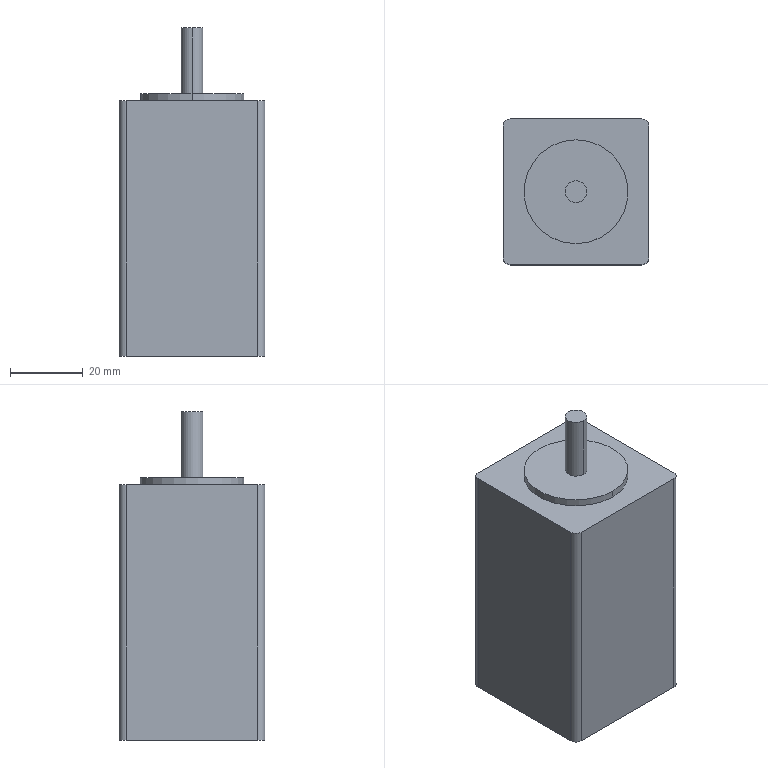Component | SolidWorks | Motor-1 | 1 solid | 16 faces | box 40 x 40 x 90 mm | volume 113537 mm3 | cylinder 8 | plane 8 | commonest cylinder face diameters 4 x4 5.952 x2 28.506 x2
build123d program:
from build123d import *

# Parameters (mm, degrees)
SKETCH1_W           = 40
SKETCH1_H           = 70
BOSS_EXTRUDE1_DEPTH = 40
FILLET1_R           = 2
BOSS_EXTRUDE2_DEPTH = 2
SKETCH3_R           = 2.976
BOSS_EXTRUDE3_DEPTH = 18


with BuildPart() as part:
    # Sketch1 → Boss-Extrude1 (new body)
    with BuildSketch(Plane.XY):
        with Locations((59.88, -78.689)):
            Rectangle(SKETCH1_W, SKETCH1_H)
    extrude(amount=BOSS_EXTRUDE1_DEPTH)

    # Fillet1
    fillet1_edges = [part.edges().sort_by_distance(p)[0] for p in [
        (79.88, -78.689, 40),
        (39.88, -78.689, 40),
        (79.88, -78.689, 0),
        (39.88, -78.689, 0),
    ]]
    fillet(fillet1_edges, radius=FILLET1_R)

    # Sketch2 → Boss-Extrude2 (add)
    with BuildSketch(Plane(origin=(0, -43.689, 0), x_dir=(1, 0, 0), z_dir=(0, 1, 0))):
        with BuildLine():
            ThreePointArc((59.88, -5.747), (45.627, -20), (59.88, -34.253))
            Line((59.88, -34.253), (59.88, -5.747))
        make_face()
        with BuildLine():
            Line((59.88, -5.747), (59.88, -34.253))
            ThreePointArc((59.88, -34.253), (69.959, -30.078), (74.133, -20))
            ThreePointArc((74.133, -20), (69.959, -9.922), (59.88, -5.747))
        make_face()
        with BuildLine():
            ThreePointArc((59.88, -5.747), (45.627, -20), (59.88, -34.253))
            Line((59.88, -34.253), (59.88, -5.747))
        make_face()
        with BuildLine():
            Line((59.88, -5.747), (59.88, -34.253))
            ThreePointArc((59.88, -34.253), (69.959, -30.078), (74.133, -20))
            ThreePointArc((74.133, -20), (69.959, -9.922), (59.88, -5.747))
        make_face()
    extrude(amount=BOSS_EXTRUDE2_DEPTH)

    # Sketch3 → Boss-Extrude3 (add)
    with BuildSketch(Plane(origin=(0, -41.689, 0), x_dir=(1, 0, 0), z_dir=(0, 1, 0))):
        with Locations(Location((59.88, -20, 0), (0, 0, 270))):
            Circle(SKETCH3_R)
    extrude(amount=BOSS_EXTRUDE3_DEPTH)


solid = part.part

# Placed as in the assembly
solid = solid.moved(Location((-11.374, -44.609, -171.311), (90, 0, 0)))
STEP:
#1=CARTESIAN_POINT('',(1.91,-2.661,-7.677));
#2=VERTEX_POINT('',#1);
#3=CARTESIAN_POINT('',(1.91,-2.426,-7.677));
#4=VERTEX_POINT('',#3);
#5=CARTESIAN_POINT('',(1.91,-2.544,-7.677));
#6=DIRECTION('',(0.,0.,1.));
#7=DIRECTION('',(0.,-1.,0.));
#8=AXIS2_PLACEMENT_3D('',#5,#6,#7);
#9=CIRCLE('',#8,0.1172);
#10=EDGE_CURVE('',#2,#4,#9,.T.);
#11=ORIENTED_EDGE('',*,*,#10,.F.);
#12=CARTESIAN_POINT('',(1.91,-2.661,-8.386));
#13=VERTEX_POINT('',#12);
#14=CARTESIAN_POINT('',(1.91,-2.661,-7.677));
#15=DIRECTION('',(0.,0.,-1.));
#16=VECTOR('',#15,39.37);
#17=LINE('',#14,#16);
#18=EDGE_CURVE('',#2,#13,#17,.T.);
#19=ORIENTED_EDGE('',*,*,#18,.T.);
#20=CARTESIAN_POINT('',(1.91,-2.426,-8.386));
#21=VERTEX_POINT('',#20);
#22=CARTESIAN_POINT('',(1.91,-2.544,-8.386));
#23=DIRECTION('',(0.,0.,1.));
#24=DIRECTION('',(0.,-1.,0.));
#25=AXIS2_PLACEMENT_3D('',#22,#23,#24);
#26=CIRCLE('',#25,0.1172);
#27=EDGE_CURVE('',#13,#21,#26,.T.);
#28=ORIENTED_EDGE('',*,*,#27,.T.);
#29=CARTESIAN_POINT('',(1.91,-2.426,-7.677));
#30=DIRECTION('',(0.,0.,-1.));
#31=VECTOR('',#30,39.37);
#32=LINE('',#29,#31);
#33=EDGE_CURVE('',#4,#21,#32,.T.);
#34=ORIENTED_EDGE('',*,*,#33,.F.);
#35=EDGE_LOOP('',(#11,#19,#28,#34));
#36=FACE_OUTER_BOUND('',#35,.T.);
#37=CARTESIAN_POINT('',(1.91,-2.544,-7.677));
#38=DIRECTION('',(0.,0.,-1.));
#39=DIRECTION('',(0.,1.,0.));
#40=AXIS2_PLACEMENT_3D('',#37,#38,#39);
#41=CYLINDRICAL_SURFACE('',#40,0.1172);
#42=ADVANCED_FACE('',(#36),#41,.T.);
#43=CARTESIAN_POINT('',(1.91,-3.105,-8.386));
#44=VERTEX_POINT('',#43);
#45=CARTESIAN_POINT('',(1.91,-1.983,-8.386));
#46=VERTEX_POINT('',#45);
#47=CARTESIAN_POINT('',(1.91,-2.544,-8.386));
#48=DIRECTION('',(0.,0.,1.));
#49=DIRECTION('',(0.,-1.,0.));
#50=AXIS2_PLACEMENT_3D('',#47,#48,#49);
#51=CIRCLE('',#50,0.5611);
#52=EDGE_CURVE('',#44,#46,#51,.T.);
#53=ORIENTED_EDGE('',*,*,#52,.F.);
#54=CARTESIAN_POINT('',(1.91,-3.105,-8.465));
#55=VERTEX_POINT('',#54);
#56=CARTESIAN_POINT('',(1.91,-3.105,-8.386));
#57=DIRECTION('',(0.,0.,-1.));
#58=VECTOR('',#57,39.37);
#59=LINE('',#56,#58);
#60=EDGE_CURVE('',#44,#55,#59,.T.);
#61=ORIENTED_EDGE('',*,*,#60,.T.);
#62=CARTESIAN_POINT('',(1.91,-1.983,-8.465));
#63=VERTEX_POINT('',#62);
#64=CARTESIAN_POINT('',(1.91,-2.544,-8.465));
#65=DIRECTION('',(0.,0.,1.));
#66=DIRECTION('',(0.,-1.,0.));
#67=AXIS2_PLACEMENT_3D('',#64,#65,#66);
#68=CIRCLE('',#67,0.5611);
#69=EDGE_CURVE('',#55,#63,#68,.T.);
#70=ORIENTED_EDGE('',*,*,#69,.T.);
#71=CARTESIAN_POINT('',(1.91,-1.983,-8.386));
#72=DIRECTION('',(0.,0.,-1.));
#73=VECTOR('',#72,39.37);
#74=LINE('',#71,#73);
#75=EDGE_CURVE('',#46,#63,#74,.T.);
#76=ORIENTED_EDGE('',*,*,#75,.F.);
#77=EDGE_LOOP('',(#53,#61,#70,#76));
#78=FACE_OUTER_BOUND('',#77,.T.);
#79=CARTESIAN_POINT('',(1.91,-2.544,-8.386));
#80=DIRECTION('',(0.,0.,-1.));
#81=DIRECTION('',(0.,1.,0.));
#82=AXIS2_PLACEMENT_3D('',#79,#80,#81);
#83=CYLINDRICAL_SURFACE('',#82,0.5611);
#84=ADVANCED_FACE('',(#78),#83,.T.);
#85=CARTESIAN_POINT('',(1.122,-3.252,-8.465));
#86=VERTEX_POINT('',#85);
#87=CARTESIAN_POINT('',(1.122,-1.835,-8.465));
#88=VERTEX_POINT('',#87);
#89=CARTESIAN_POINT('',(1.122,-3.331,-8.465));
#90=DIRECTION('',(0.,1.,0.));
#91=VECTOR('',#90,39.37);
#92=LINE('',#89,#91);
#93=EDGE_CURVE('',#86,#88,#92,.T.);
#94=ORIENTED_EDGE('',*,*,#93,.T.);
#95=CARTESIAN_POINT('',(1.122,-1.835,-11.22));
#96=VERTEX_POINT('',#95);
#97=CARTESIAN_POINT('',(1.122,-1.835,-8.465));
#98=DIRECTION('',(0.,0.,-1.));
#99=VECTOR('',#98,39.37);
#100=LINE('',#97,#99);
#101=EDGE_CURVE('',#88,#96,#100,.T.);
#102=ORIENTED_EDGE('',*,*,#101,.T.);
#103=CARTESIAN_POINT('',(1.122,-3.252,-11.22));
#104=VERTEX_POINT('',#103);
#105=CARTESIAN_POINT('',(1.122,-3.331,-11.22));
#106=DIRECTION('',(0.,1.,0.));
#107=VECTOR('',#106,39.37);
#108=LINE('',#105,#107);
#109=EDGE_CURVE('',#104,#96,#108,.T.);
#110=ORIENTED_EDGE('',*,*,#109,.F.);
#111=CARTESIAN_POINT('',(1.122,-3.252,-8.465));
#112=DIRECTION('',(-0.,0.,1.));
#113=VECTOR('',#112,39.37);
#114=LINE('',#111,#113);
#115=EDGE_CURVE('',#104,#86,#114,.T.);
#116=ORIENTED_EDGE('',*,*,#115,.T.);
#117=EDGE_LOOP('',(#94,#102,#110,#116));
#118=FACE_OUTER_BOUND('',#117,.T.);
#119=CARTESIAN_POINT('',(1.122,-3.331,-8.465));
#120=DIRECTION('',(1.,0.,0.));
#121=DIRECTION('',(-0.,0.,1.));
#122=AXIS2_PLACEMENT_3D('',#119,#120,#121);
#123=PLANE('',#122);
#124=ADVANCED_FACE('',(#118),#123,.F.);
#125=CARTESIAN_POINT('',(1.201,-1.756,-11.22));
#126=VERTEX_POINT('',#125);
#127=CARTESIAN_POINT('',(2.618,-1.756,-11.22));
#128=VERTEX_POINT('',#127);
#129=CARTESIAN_POINT('',(1.122,-1.756,-11.22));
#130=DIRECTION('',(1.,0.,0.));
#131=VECTOR('',#130,39.37);
#132=LINE('',#129,#131);
#133=EDGE_CURVE('',#126,#128,#132,.T.);
#134=ORIENTED_EDGE('',*,*,#133,.T.);
#135=CARTESIAN_POINT('',(2.697,-1.835,-11.22));
#136=VERTEX_POINT('',#135);
#137=CARTESIAN_POINT('',(2.618,-1.835,-11.22));
#138=DIRECTION('',(0.,0.,-1.));
#139=DIRECTION('',(0.,-1.,0.));
#140=AXIS2_PLACEMENT_3D('',#137,#138,#139);
#141=CIRCLE('',#140,0.07874);
#142=EDGE_CURVE('',#128,#136,#141,.T.);
#143=ORIENTED_EDGE('',*,*,#142,.T.);
#144=CARTESIAN_POINT('',(2.697,-3.252,-11.22));
#145=VERTEX_POINT('',#144);
#146=CARTESIAN_POINT('',(2.697,-3.331,-11.22));
#147=DIRECTION('',(0.,1.,0.));
#148=VECTOR('',#147,39.37);
#149=LINE('',#146,#148);
#150=EDGE_CURVE('',#145,#136,#149,.T.);
#151=ORIENTED_EDGE('',*,*,#150,.F.);
#152=CARTESIAN_POINT('',(2.618,-3.331,-11.22));
#153=VERTEX_POINT('',#152);
#154=CARTESIAN_POINT('',(2.618,-3.252,-11.22));
#155=DIRECTION('',(0.,0.,-1.));
#156=DIRECTION('',(0.,-1.,0.));
#157=AXIS2_PLACEMENT_3D('',#154,#155,#156);
#158=CIRCLE('',#157,0.07874);
#159=EDGE_CURVE('',#145,#153,#158,.T.);
#160=ORIENTED_EDGE('',*,*,#159,.T.);
#161=CARTESIAN_POINT('',(1.201,-3.331,-11.22));
#162=VERTEX_POINT('',#161);
#163=CARTESIAN_POINT('',(1.122,-3.331,-11.22));
#164=DIRECTION('',(1.,0.,0.));
#165=VECTOR('',#164,39.37);
#166=LINE('',#163,#165);
#167=EDGE_CURVE('',#162,#153,#166,.T.);
#168=ORIENTED_EDGE('',*,*,#167,.F.);
#169=CARTESIAN_POINT('',(1.201,-3.252,-11.22));
#170=DIRECTION('',(0.,0.,-1.));
#171=DIRECTION('',(0.,-1.,0.));
#172=AXIS2_PLACEMENT_3D('',#169,#170,#171);
#173=CIRCLE('',#172,0.07874);
#174=EDGE_CURVE('',#162,#104,#173,.T.);
#175=ORIENTED_EDGE('',*,*,#174,.T.);
#176=ORIENTED_EDGE('',*,*,#109,.T.);
#177=CARTESIAN_POINT('',(1.201,-1.835,-11.22));
#178=DIRECTION('',(0.,0.,-1.));
#179=DIRECTION('',(0.,-1.,0.));
#180=AXIS2_PLACEMENT_3D('',#177,#178,#179);
#181=CIRCLE('',#180,0.07874);
#182=EDGE_CURVE('',#96,#126,#181,.T.);
#183=ORIENTED_EDGE('',*,*,#182,.T.);
#184=EDGE_LOOP('',(#134,#143,#151,#160,#168,#175,#176,#183));
#185=FACE_OUTER_BOUND('',#184,.T.);
#186=CARTESIAN_POINT('',(1.122,-3.331,-11.22));
#187=DIRECTION('',(0.,0.,1.));
#188=DIRECTION('',(0.,-1.,0.));
#189=AXIS2_PLACEMENT_3D('',#186,#187,#188);
#190=PLANE('',#189);
#191=ADVANCED_FACE('',(#185),#190,.F.);
#192=ORIENTED_EDGE('',*,*,#150,.T.);
#193=CARTESIAN_POINT('',(2.697,-1.835,-8.465));
#194=VERTEX_POINT('',#193);
#195=CARTESIAN_POINT('',(2.697,-1.835,-8.465));
#196=DIRECTION('',(0.,0.,1.));
#197=VECTOR('',#196,39.37);
#198=LINE('',#195,#197);
#199=EDGE_CURVE('',#136,#194,#198,.T.);
#200=ORIENTED_EDGE('',*,*,#199,.T.);
#201=CARTESIAN_POINT('',(2.697,-3.252,-8.465));
#202=VERTEX_POINT('',#201);
#203=CARTESIAN_POINT('',(2.697,-3.331,-8.465));
#204=DIRECTION('',(0.,1.,0.));
#205=VECTOR('',#204,39.37);
#206=LINE('',#203,#205);
#207=EDGE_CURVE('',#202,#194,#206,.T.);
#208=ORIENTED_EDGE('',*,*,#207,.F.);
#209=CARTESIAN_POINT('',(2.697,-3.252,-11.22));
#210=DIRECTION('',(0.,0.,-1.));
#211=VECTOR('',#210,39.37);
#212=LINE('',#209,#211);
#213=EDGE_CURVE('',#202,#145,#212,.T.);
#214=ORIENTED_EDGE('',*,*,#213,.T.);
#215=EDGE_LOOP('',(#192,#200,#208,#214));
#216=FACE_OUTER_BOUND('',#215,.T.);
#217=CARTESIAN_POINT('',(2.697,-3.331,-8.465));
#218=DIRECTION('',(-1.,0.,0.));
#219=DIRECTION('',(0.,-1.,0.));
#220=AXIS2_PLACEMENT_3D('',#217,#218,#219);
#221=PLANE('',#220);
#222=ADVANCED_FACE('',(#216),#221,.F.);
#223=CARTESIAN_POINT('',(1.91,-2.544,-8.465));
#224=DIRECTION('',(0.,0.,1.));
#225=DIRECTION('',(0.,-1.,0.));
#226=AXIS2_PLACEMENT_3D('',#223,#224,#225);
#227=CIRCLE('',#226,0.5611);
#228=EDGE_CURVE('',#63,#55,#227,.T.);
#229=ORIENTED_EDGE('',*,*,#228,.F.);
#230=ORIENTED_EDGE('',*,*,#69,.F.);
#231=EDGE_LOOP('',(#229,#230));
#232=FACE_BOUND('',#231,.T.);
#233=ORIENTED_EDGE('',*,*,#207,.T.);
#234=CARTESIAN_POINT('',(2.618,-1.756,-8.465));
#235=VERTEX_POINT('',#234);
#236=CARTESIAN_POINT('',(2.618,-1.835,-8.465));
#237=DIRECTION('',(0.,0.,1.));
#238=DIRECTION('',(0.,1.,0.));
#239=AXIS2_PLACEMENT_3D('',#236,#237,#238);
#240=CIRCLE('',#239,0.07874);
#241=EDGE_CURVE('',#194,#235,#240,.T.);
#242=ORIENTED_EDGE('',*,*,#241,.T.);
#243=CARTESIAN_POINT('',(1.201,-1.756,-8.465));
#244=VERTEX_POINT('',#243);
#245=CARTESIAN_POINT('',(1.122,-1.756,-8.465));
#246=DIRECTION('',(-1.,0.,0.));
#247=VECTOR('',#246,39.37);
#248=LINE('',#245,#247);
#249=EDGE_CURVE('',#235,#244,#248,.T.);
#250=ORIENTED_EDGE('',*,*,#249,.T.);
#251=CARTESIAN_POINT('',(1.201,-1.835,-8.465));
#252=DIRECTION('',(0.,0.,1.));
#253=DIRECTION('',(0.,1.,0.));
#254=AXIS2_PLACEMENT_3D('',#251,#252,#253);
#255=CIRCLE('',#254,0.07874);
#256=EDGE_CURVE('',#244,#88,#255,.T.);
#257=ORIENTED_EDGE('',*,*,#256,.T.);
#258=ORIENTED_EDGE('',*,*,#93,.F.);
#259=CARTESIAN_POINT('',(1.201,-3.331,-8.465));
#260=VERTEX_POINT('',#259);
#261=CARTESIAN_POINT('',(1.201,-3.252,-8.465));
#262=DIRECTION('',(0.,0.,1.));
#263=DIRECTION('',(0.,1.,0.));
#264=AXIS2_PLACEMENT_3D('',#261,#262,#263);
#265=CIRCLE('',#264,0.07874);
#266=EDGE_CURVE('',#86,#260,#265,.T.);
#267=ORIENTED_EDGE('',*,*,#266,.T.);
#268=CARTESIAN_POINT('',(2.618,-3.331,-8.465));
#269=VERTEX_POINT('',#268);
#270=CARTESIAN_POINT('',(1.122,-3.331,-8.465));
#271=DIRECTION('',(-1.,0.,0.));
#272=VECTOR('',#271,39.37);
#273=LINE('',#270,#272);
#274=EDGE_CURVE('',#269,#260,#273,.T.);
#275=ORIENTED_EDGE('',*,*,#274,.F.);
#276=CARTESIAN_POINT('',(2.618,-3.252,-8.465));
#277=DIRECTION('',(0.,0.,1.));
#278=DIRECTION('',(0.,1.,0.));
#279=AXIS2_PLACEMENT_3D('',#276,#277,#278);
#280=CIRCLE('',#279,0.07874);
#281=EDGE_CURVE('',#269,#202,#280,.T.);
#282=ORIENTED_EDGE('',*,*,#281,.T.);
#283=EDGE_LOOP('',(#233,#242,#250,#257,#258,#267,#275,#282));
#284=FACE_OUTER_BOUND('',#283,.T.);
#285=CARTESIAN_POINT('',(1.122,-3.331,-8.465));
#286=DIRECTION('',(0.,0.,-1.));
#287=DIRECTION('',(0.,1.,0.));
#288=AXIS2_PLACEMENT_3D('',#285,#286,#287);
#289=PLANE('',#288);
#290=ADVANCED_FACE('',(#232,#284),#289,.F.);
#291=ORIENTED_EDGE('',*,*,#274,.T.);
#292=CARTESIAN_POINT('',(1.201,-3.331,-11.22));
#293=DIRECTION('',(0.,0.,-1.));
#294=VECTOR('',#293,39.37);
#295=LINE('',#292,#294);
#296=EDGE_CURVE('',#260,#162,#295,.T.);
#297=ORIENTED_EDGE('',*,*,#296,.T.);
#298=ORIENTED_EDGE('',*,*,#167,.T.);
#299=CARTESIAN_POINT('',(2.618,-3.331,-8.465));
#300=DIRECTION('',(0.,0.,1.));
#301=VECTOR('',#300,39.37);
#302=LINE('',#299,#301);
#303=EDGE_CURVE('',#153,#269,#302,.T.);
#304=ORIENTED_EDGE('',*,*,#303,.T.);
#305=EDGE_LOOP('',(#291,#297,#298,#304));
#306=FACE_OUTER_BOUND('',#305,.T.);
#307=CARTESIAN_POINT('',(-0.4478,-3.331,-6.745));
#308=DIRECTION('',(0.,-1.,0.));
#309=DIRECTION('',(1.,0.,0.));
#310=AXIS2_PLACEMENT_3D('',#307,#308,#309);
#311=PLANE('',#310);
#312=ADVANCED_FACE('',(#306),#311,.T.);
#313=ORIENTED_EDGE('',*,*,#249,.F.);
#314=CARTESIAN_POINT('',(2.618,-1.756,-6.745));
#315=DIRECTION('',(0.,0.,-1.));
#316=VECTOR('',#315,39.37);
#317=LINE('',#314,#316);
#318=EDGE_CURVE('',#235,#128,#317,.T.);
#319=ORIENTED_EDGE('',*,*,#318,.T.);
#320=ORIENTED_EDGE('',*,*,#133,.F.);
#321=CARTESIAN_POINT('',(1.201,-1.756,-6.745));
#322=DIRECTION('',(-0.,0.,1.));
#323=VECTOR('',#322,39.37);
#324=LINE('',#321,#323);
#325=EDGE_CURVE('',#126,#244,#324,.T.);
#326=ORIENTED_EDGE('',*,*,#325,.T.);
#327=EDGE_LOOP('',(#313,#319,#320,#326));
#328=FACE_OUTER_BOUND('',#327,.T.);
#329=CARTESIAN_POINT('',(-0.4478,-1.756,-6.745));
#330=DIRECTION('',(0.,-1.,0.));
#331=DIRECTION('',(1.,0.,0.));
#332=AXIS2_PLACEMENT_3D('',#329,#330,#331);
#333=PLANE('',#332);
#334=ADVANCED_FACE('',(#328),#333,.F.);
#335=ORIENTED_EDGE('',*,*,#142,.F.);
#336=ORIENTED_EDGE('',*,*,#318,.F.);
#337=ORIENTED_EDGE('',*,*,#241,.F.);
#338=ORIENTED_EDGE('',*,*,#199,.F.);
#339=EDGE_LOOP('',(#335,#336,#337,#338));
#340=FACE_OUTER_BOUND('',#339,.T.);
#341=CARTESIAN_POINT('',(2.618,-1.835,-8.465));
#342=DIRECTION('',(0.,0.,1.));
#343=DIRECTION('',(0.,-1.,0.));
#344=AXIS2_PLACEMENT_3D('',#341,#342,#343);
#345=CYLINDRICAL_SURFACE('',#344,0.07874);
#346=ADVANCED_FACE('',(#340),#345,.T.);
#347=ORIENTED_EDGE('',*,*,#256,.F.);
#348=ORIENTED_EDGE('',*,*,#325,.F.);
#349=ORIENTED_EDGE('',*,*,#182,.F.);
#350=ORIENTED_EDGE('',*,*,#101,.F.);
#351=EDGE_LOOP('',(#347,#348,#349,#350));
#352=FACE_OUTER_BOUND('',#351,.T.);
#353=CARTESIAN_POINT('',(1.201,-1.835,-8.465));
#354=DIRECTION('',(0.,0.,-1.));
#355=DIRECTION('',(1.,0.,0.));
#356=AXIS2_PLACEMENT_3D('',#353,#354,#355);
#357=CYLINDRICAL_SURFACE('',#356,0.07874);
#358=ADVANCED_FACE('',(#352),#357,.T.);
#359=ORIENTED_EDGE('',*,*,#266,.F.);
#360=ORIENTED_EDGE('',*,*,#115,.F.);
#361=ORIENTED_EDGE('',*,*,#174,.F.);
#362=ORIENTED_EDGE('',*,*,#296,.F.);
#363=EDGE_LOOP('',(#359,#360,#361,#362));
#364=FACE_OUTER_BOUND('',#363,.T.);
#365=CARTESIAN_POINT('',(1.201,-3.252,-6.745));
#366=DIRECTION('',(-0.,0.,1.));
#367=DIRECTION('',(-1.,0.,0.));
#368=AXIS2_PLACEMENT_3D('',#365,#366,#367);
#369=CYLINDRICAL_SURFACE('',#368,0.07874);
#370=ADVANCED_FACE('',(#364),#369,.T.);
#371=ORIENTED_EDGE('',*,*,#159,.F.);
#372=ORIENTED_EDGE('',*,*,#213,.F.);
#373=ORIENTED_EDGE('',*,*,#281,.F.);
#374=ORIENTED_EDGE('',*,*,#303,.F.);
#375=EDGE_LOOP('',(#371,#372,#373,#374));
#376=FACE_OUTER_BOUND('',#375,.T.);
#377=CARTESIAN_POINT('',(2.618,-3.252,-6.745));
#378=DIRECTION('',(0.,0.,-1.));
#379=DIRECTION('',(0.,1.,0.));
#380=AXIS2_PLACEMENT_3D('',#377,#378,#379);
#381=CYLINDRICAL_SURFACE('',#380,0.07874);
#382=ADVANCED_FACE('',(#376),#381,.T.);
#383=ORIENTED_EDGE('',*,*,#60,.F.);
#384=CARTESIAN_POINT('',(1.91,-2.544,-8.386));
#385=DIRECTION('',(0.,0.,1.));
#386=DIRECTION('',(0.,-1.,0.));
#387=AXIS2_PLACEMENT_3D('',#384,#385,#386);
#388=CIRCLE('',#387,0.5611);
#389=EDGE_CURVE('',#46,#44,#388,.T.);
#390=ORIENTED_EDGE('',*,*,#389,.F.);
#391=ORIENTED_EDGE('',*,*,#75,.T.);
#392=ORIENTED_EDGE('',*,*,#228,.T.);
#393=EDGE_LOOP('',(#383,#390,#391,#392));
#394=FACE_OUTER_BOUND('',#393,.T.);
#395=CARTESIAN_POINT('',(1.91,-2.544,-8.386));
#396=DIRECTION('',(0.,0.,-1.));
#397=DIRECTION('',(0.,1.,0.));
#398=AXIS2_PLACEMENT_3D('',#395,#396,#397);
#399=CYLINDRICAL_SURFACE('',#398,0.5611);
#400=ADVANCED_FACE('',(#394),#399,.T.);
#401=CARTESIAN_POINT('',(1.91,-2.544,-8.386));
#402=DIRECTION('',(0.,0.,1.));
#403=DIRECTION('',(0.,-1.,0.));
#404=AXIS2_PLACEMENT_3D('',#401,#402,#403);
#405=CIRCLE('',#404,0.1172);
#406=EDGE_CURVE('',#21,#13,#405,.T.);
#407=ORIENTED_EDGE('',*,*,#406,.F.);
#408=ORIENTED_EDGE('',*,*,#27,.F.);
#409=EDGE_LOOP('',(#407,#408));
#410=FACE_BOUND('',#409,.T.);
#411=ORIENTED_EDGE('',*,*,#389,.T.);
#412=ORIENTED_EDGE('',*,*,#52,.T.);
#413=EDGE_LOOP('',(#411,#412));
#414=FACE_OUTER_BOUND('',#413,.T.);
#415=CARTESIAN_POINT('',(-0.4478,-1.756,-8.386));
#416=DIRECTION('',(0.,0.,1.));
#417=DIRECTION('',(0.,-1.,0.));
#418=AXIS2_PLACEMENT_3D('',#415,#416,#417);
#419=PLANE('',#418);
#420=ADVANCED_FACE('',(#410,#414),#419,.T.);
#421=ORIENTED_EDGE('',*,*,#18,.F.);
#422=CARTESIAN_POINT('',(1.91,-2.544,-7.677));
#423=DIRECTION('',(0.,0.,1.));
#424=DIRECTION('',(0.,-1.,0.));
#425=AXIS2_PLACEMENT_3D('',#422,#423,#424);
#426=CIRCLE('',#425,0.1172);
#427=EDGE_CURVE('',#4,#2,#426,.T.);
#428=ORIENTED_EDGE('',*,*,#427,.F.);
#429=ORIENTED_EDGE('',*,*,#33,.T.);
#430=ORIENTED_EDGE('',*,*,#406,.T.);
#431=EDGE_LOOP('',(#421,#428,#429,#430));
#432=FACE_OUTER_BOUND('',#431,.T.);
#433=CARTESIAN_POINT('',(1.91,-2.544,-7.677));
#434=DIRECTION('',(0.,0.,-1.));
#435=DIRECTION('',(0.,1.,0.));
#436=AXIS2_PLACEMENT_3D('',#433,#434,#435);
#437=CYLINDRICAL_SURFACE('',#436,0.1172);
#438=ADVANCED_FACE('',(#432),#437,.T.);
#439=ORIENTED_EDGE('',*,*,#427,.T.);
#440=ORIENTED_EDGE('',*,*,#10,.T.);
#441=EDGE_LOOP('',(#439,#440));
#442=FACE_OUTER_BOUND('',#441,.T.);
#443=CARTESIAN_POINT('',(1.91,-2.544,-7.677));
#444=DIRECTION('',(0.,0.,1.));
#445=DIRECTION('',(0.,-1.,0.));
#446=AXIS2_PLACEMENT_3D('',#443,#444,#445);
#447=PLANE('',#446);
#448=ADVANCED_FACE('',(#442),#447,.T.);
#449=CLOSED_SHELL('',(#42,#84,#124,#191,#222,#290,#312,#334,#346,#358,#370,#382,#400,#420,#438,#448));
#450=MANIFOLD_SOLID_BREP('',#449);
#451=CARTESIAN_POINT('',(0.,0.,0.));
#452=DIRECTION('',(0.,0.,1.));
#453=DIRECTION('',(1.,0.,0.));
#454=AXIS2_PLACEMENT_3D('',#451,#452,#453);
#455=(LENGTH_UNIT()NAMED_UNIT(*)SI_UNIT($,.METRE.));
#456=LENGTH_MEASURE_WITH_UNIT(LENGTH_MEASURE(0.0254),#455);
#457=DIMENSIONAL_EXPONENTS(1.,0.,0.,0.,0.,0.,0.);
#458=(CONVERSION_BASED_UNIT('',#456)LENGTH_UNIT()NAMED_UNIT(#457));
#459=UNCERTAINTY_MEASURE_WITH_UNIT(LENGTH_MEASURE(0.00001),#458,'','');
#460=(NAMED_UNIT(*)PLANE_ANGLE_UNIT()SI_UNIT($,.RADIAN.));
#461=(NAMED_UNIT(*)SI_UNIT($,.STERADIAN.)SOLID_ANGLE_UNIT());
#462=(GEOMETRIC_REPRESENTATION_CONTEXT(3)GLOBAL_UNCERTAINTY_ASSIGNED_CONTEXT((#459))GLOBAL_UNIT_ASSIGNED_CONTEXT((#458,#460,#461))REPRESENTATION_CONTEXT('',''));
#463=ADVANCED_BREP_SHAPE_REPRESENTATION('',(#450,#454),#462);
#464=COLOUR_RGB('',0.7922,0.8196,0.9333);
#465=FILL_AREA_STYLE_COLOUR('',#464);
#466=FILL_AREA_STYLE('',(#465));
#467=SURFACE_STYLE_FILL_AREA(#466);
#468=SURFACE_SIDE_STYLE('',(#467));
#469=SURFACE_STYLE_USAGE(.BOTH.,#468);
#470=PRESENTATION_STYLE_ASSIGNMENT((#469));
#471=STYLED_ITEM('',(#470),#450);
#472=PRESENTATION_LAYER_ASSIGNMENT('','',(#471));
#473=(LENGTH_UNIT()NAMED_UNIT(*)SI_UNIT($,.METRE.));
#474=LENGTH_MEASURE_WITH_UNIT(LENGTH_MEASURE(0.0254),#473);
#475=DIMENSIONAL_EXPONENTS(1.,0.,0.,0.,0.,0.,0.);
#476=(CONVERSION_BASED_UNIT('',#474)LENGTH_UNIT()NAMED_UNIT(#475));
#477=UNCERTAINTY_MEASURE_WITH_UNIT(LENGTH_MEASURE(0.00001),#476,'','');
#478=(NAMED_UNIT(*)PLANE_ANGLE_UNIT()SI_UNIT($,.RADIAN.));
#479=(NAMED_UNIT(*)SI_UNIT($,.STERADIAN.)SOLID_ANGLE_UNIT());
#480=(GEOMETRIC_REPRESENTATION_CONTEXT(3)GLOBAL_UNCERTAINTY_ASSIGNED_CONTEXT((#477))GLOBAL_UNIT_ASSIGNED_CONTEXT((#476,#478,#479))REPRESENTATION_CONTEXT('',''));
#481=MECHANICAL_DESIGN_GEOMETRIC_PRESENTATION_REPRESENTATION('',(#471),#480);